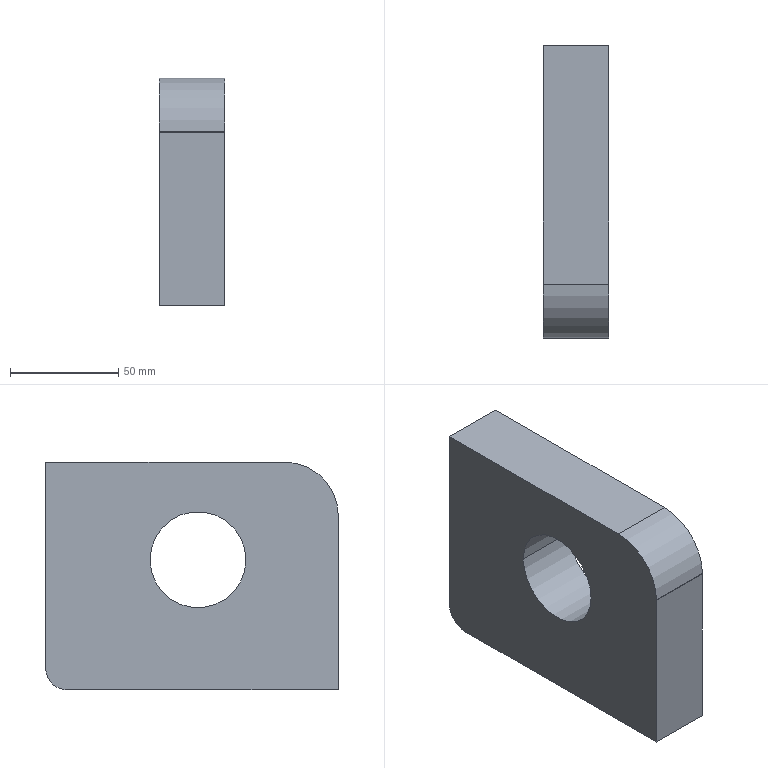Component | SolidWorks | ForkLug-1 | 1 solid | 11 faces | box 30 x 134.85 x 105 mm | volume 374154 mm3 | plane 6 | cylinder 5 | commonest cylinder face diameters 44.2 x2 49.483 x2 20 x1 | material Q235
build123d program:
from build123d import *

# Parameters (mm, degrees)
SKETCH1_R           = 22.1
BOSS_EXTRUDE1_DEPTH = 30


with BuildPart() as part:
    # Sketch1 → Boss-Extrude1 (new body)
    with BuildSketch(Plane.XY):
        with BuildLine():
            Line((3.712, 96.226), (103.712, 96.226))
            Line((103.712, 96.226), (113.712, 96.226))
            Line((113.712, 96.226), (113.712, 1.226))
            ThreePointArc((113.712, 1.226), (110.783, -5.845), (103.712, -8.774))
            Line((103.712, -8.774), (93.712, -8.774))
            Line((93.712, -8.774), (-21.136, -8.774))
            Line((-21.136, -8.774), (-21.136, 71.226))
            ThreePointArc((-21.136, 71.226), (-13.944, 88.926), (3.712, 96.226))
        make_face()
        with Locations((43.545, 51.226)):
            Circle(SKETCH1_R, mode=Mode.SUBTRACT)
    extrude(amount=BOSS_EXTRUDE1_DEPTH)


solid = part.part

# Placed as in the assembly
solid = solid.moved(Location((-1146.164, 1663.762, 2829.479), (90, 90, 0)))
STEP:
#1=COLOUR_RGB('',0.7922,0.8196,0.9333);
#2=FILL_AREA_STYLE_COLOUR('',#1);
#3=FILL_AREA_STYLE('',(#2));
#4=SURFACE_STYLE_FILL_AREA(#3);
#5=SURFACE_SIDE_STYLE('',(#4));
#6=SURFACE_STYLE_USAGE(.BOTH.,#5);
#7=PRESENTATION_STYLE_ASSIGNMENT((#6));
#8=CARTESIAN_POINT('',(-43.943,66.347,113.414));
#9=VERTEX_POINT('',#8);
#10=CARTESIAN_POINT('',(-43.943,68.087,113.414));
#11=VERTEX_POINT('',#10);
#12=CARTESIAN_POINT('',(-43.943,67.217,113.414));
#13=DIRECTION('',(1.,0.,-0.));
#14=DIRECTION('',(0.,1.,0.));
#15=AXIS2_PLACEMENT_3D('',#12,#13,#14);
#16=CIRCLE('',#15,0.8701);
#17=EDGE_CURVE('',#9,#11,#16,.T.);
#18=ORIENTED_EDGE('',*,*,#17,.T.);
#19=CARTESIAN_POINT('',(-45.125,68.087,113.414));
#20=VERTEX_POINT('',#19);
#21=CARTESIAN_POINT('',(-43.943,68.087,113.414));
#22=DIRECTION('',(-1.,-0.,0.));
#23=VECTOR('',#22,39.37);
#24=LINE('',#21,#23);
#25=EDGE_CURVE('',#11,#20,#24,.T.);
#26=ORIENTED_EDGE('',*,*,#25,.T.);
#27=CARTESIAN_POINT('',(-45.125,66.347,113.414));
#28=VERTEX_POINT('',#27);
#29=CARTESIAN_POINT('',(-45.125,67.217,113.414));
#30=DIRECTION('',(1.,0.,-0.));
#31=DIRECTION('',(0.,1.,0.));
#32=AXIS2_PLACEMENT_3D('',#29,#30,#31);
#33=CIRCLE('',#32,0.8701);
#34=EDGE_CURVE('',#28,#20,#33,.T.);
#35=ORIENTED_EDGE('',*,*,#34,.F.);
#36=CARTESIAN_POINT('',(-43.943,66.347,113.414));
#37=DIRECTION('',(-1.,-0.,0.));
#38=VECTOR('',#37,39.37);
#39=LINE('',#36,#38);
#40=EDGE_CURVE('',#9,#28,#39,.T.);
#41=ORIENTED_EDGE('',*,*,#40,.F.);
#42=EDGE_LOOP('',(#18,#26,#35,#41));
#43=FACE_OUTER_BOUND('',#42,.T.);
#44=CARTESIAN_POINT('',(-43.943,67.217,113.414));
#45=DIRECTION('',(-1.,-0.,0.));
#46=DIRECTION('',(0.,-1.,0.));
#47=AXIS2_PLACEMENT_3D('',#44,#45,#46);
#48=CYLINDRICAL_SURFACE('',#47,0.8701);
#49=ADVANCED_FACE('',(#43),#48,.F.);
#50=CARTESIAN_POINT('',(-43.943,64.67,114.211));
#51=VERTEX_POINT('',#50);
#52=CARTESIAN_POINT('',(-43.943,64.67,114.201));
#53=VERTEX_POINT('',#52);
#54=CARTESIAN_POINT('',(-43.943,65.644,114.211));
#55=DIRECTION('',(1.,0.,-0.));
#56=DIRECTION('',(0.,1.,0.));
#57=AXIS2_PLACEMENT_3D('',#54,#55,#56);
#58=CIRCLE('',#57,0.9741);
#59=EDGE_CURVE('',#51,#53,#58,.T.);
#60=ORIENTED_EDGE('',*,*,#59,.F.);
#61=CARTESIAN_POINT('',(-45.125,64.67,114.211));
#62=VERTEX_POINT('',#61);
#63=CARTESIAN_POINT('',(-43.943,64.67,114.211));
#64=DIRECTION('',(-1.,-0.,0.));
#65=VECTOR('',#64,39.37);
#66=LINE('',#63,#65);
#67=EDGE_CURVE('',#51,#62,#66,.T.);
#68=ORIENTED_EDGE('',*,*,#67,.T.);
#69=CARTESIAN_POINT('',(-45.125,64.67,114.201));
#70=VERTEX_POINT('',#69);
#71=CARTESIAN_POINT('',(-45.125,65.644,114.211));
#72=DIRECTION('',(1.,0.,-0.));
#73=DIRECTION('',(0.,1.,0.));
#74=AXIS2_PLACEMENT_3D('',#71,#72,#73);
#75=CIRCLE('',#74,0.9741);
#76=EDGE_CURVE('',#62,#70,#75,.T.);
#77=ORIENTED_EDGE('',*,*,#76,.T.);
#78=CARTESIAN_POINT('',(-43.943,64.67,114.201));
#79=DIRECTION('',(-1.,-0.,0.));
#80=VECTOR('',#79,39.37);
#81=LINE('',#78,#80);
#82=EDGE_CURVE('',#53,#70,#81,.T.);
#83=ORIENTED_EDGE('',*,*,#82,.F.);
#84=EDGE_LOOP('',(#60,#68,#77,#83));
#85=FACE_OUTER_BOUND('',#84,.T.);
#86=CARTESIAN_POINT('',(-43.943,65.644,114.211));
#87=DIRECTION('',(-1.,-0.,0.));
#88=DIRECTION('',(0.,-1.,0.));
#89=AXIS2_PLACEMENT_3D('',#86,#87,#88);
#90=CYLINDRICAL_SURFACE('',#89,0.9741);
#91=ADVANCED_FACE('',(#85),#90,.T.);
#92=CARTESIAN_POINT('',(-43.943,69.586,111.051));
#93=VERTEX_POINT('',#92);
#94=CARTESIAN_POINT('',(-43.943,69.979,111.445));
#95=VERTEX_POINT('',#94);
#96=CARTESIAN_POINT('',(-43.943,69.586,111.445));
#97=DIRECTION('',(1.,0.,-0.));
#98=DIRECTION('',(0.,1.,0.));
#99=AXIS2_PLACEMENT_3D('',#96,#97,#98);
#100=CIRCLE('',#99,0.3937);
#101=EDGE_CURVE('',#93,#95,#100,.T.);
#102=ORIENTED_EDGE('',*,*,#101,.T.);
#103=CARTESIAN_POINT('',(-43.943,69.979,115.185));
#104=VERTEX_POINT('',#103);
#105=CARTESIAN_POINT('',(-43.943,69.979,115.185));
#106=DIRECTION('',(0.,-0.,1.));
#107=VECTOR('',#106,39.37);
#108=LINE('',#105,#107);
#109=EDGE_CURVE('',#95,#104,#108,.T.);
#110=ORIENTED_EDGE('',*,*,#109,.T.);
#111=CARTESIAN_POINT('',(-43.943,65.649,115.185));
#112=VERTEX_POINT('',#111);
#113=CARTESIAN_POINT('',(-43.943,69.586,115.185));
#114=DIRECTION('',(0.,-1.,0.));
#115=VECTOR('',#114,39.37);
#116=LINE('',#113,#115);
#117=EDGE_CURVE('',#104,#112,#116,.T.);
#118=ORIENTED_EDGE('',*,*,#117,.T.);
#119=CARTESIAN_POINT('',(-43.943,65.644,114.211));
#120=DIRECTION('',(1.,0.,-0.));
#121=DIRECTION('',(0.,1.,0.));
#122=AXIS2_PLACEMENT_3D('',#119,#120,#121);
#123=CIRCLE('',#122,0.9741);
#124=EDGE_CURVE('',#112,#51,#123,.T.);
#125=ORIENTED_EDGE('',*,*,#124,.T.);
#126=ORIENTED_EDGE('',*,*,#59,.T.);
#127=CARTESIAN_POINT('',(-43.943,64.67,111.051));
#128=VERTEX_POINT('',#127);
#129=CARTESIAN_POINT('',(-43.943,64.67,114.201));
#130=DIRECTION('',(-0.,-0.,-1.));
#131=VECTOR('',#130,39.37);
#132=LINE('',#129,#131);
#133=EDGE_CURVE('',#53,#128,#132,.T.);
#134=ORIENTED_EDGE('',*,*,#133,.T.);
#135=CARTESIAN_POINT('',(-43.943,64.67,111.051));
#136=DIRECTION('',(-0.,1.,0.));
#137=VECTOR('',#136,39.37);
#138=LINE('',#135,#137);
#139=EDGE_CURVE('',#128,#93,#138,.T.);
#140=ORIENTED_EDGE('',*,*,#139,.T.);
#141=EDGE_LOOP('',(#102,#110,#118,#125,#126,#134,#140));
#142=FACE_OUTER_BOUND('',#141,.T.);
#143=ORIENTED_EDGE('',*,*,#17,.F.);
#144=CARTESIAN_POINT('',(-43.943,67.217,113.414));
#145=DIRECTION('',(1.,0.,-0.));
#146=DIRECTION('',(0.,1.,0.));
#147=AXIS2_PLACEMENT_3D('',#144,#145,#146);
#148=CIRCLE('',#147,0.8701);
#149=EDGE_CURVE('',#11,#9,#148,.T.);
#150=ORIENTED_EDGE('',*,*,#149,.F.);
#151=EDGE_LOOP('',(#143,#150));
#152=FACE_BOUND('',#151,.T.);
#153=CARTESIAN_POINT('',(-43.943,69.586,111.445));
#154=DIRECTION('',(1.,0.,-0.));
#155=DIRECTION('',(-0.,1.,0.));
#156=AXIS2_PLACEMENT_3D('',#153,#154,#155);
#157=PLANE('',#156);
#158=ADVANCED_FACE('',(#142,#152),#157,.T.);
#159=CARTESIAN_POINT('',(-45.125,69.586,111.051));
#160=VERTEX_POINT('',#159);
#161=CARTESIAN_POINT('',(-45.125,69.979,111.445));
#162=VERTEX_POINT('',#161);
#163=CARTESIAN_POINT('',(-45.125,69.586,111.445));
#164=DIRECTION('',(1.,0.,-0.));
#165=DIRECTION('',(0.,1.,0.));
#166=AXIS2_PLACEMENT_3D('',#163,#164,#165);
#167=CIRCLE('',#166,0.3937);
#168=EDGE_CURVE('',#160,#162,#167,.T.);
#169=ORIENTED_EDGE('',*,*,#168,.F.);
#170=CARTESIAN_POINT('',(-45.125,64.67,111.051));
#171=VERTEX_POINT('',#170);
#172=CARTESIAN_POINT('',(-45.125,69.192,111.051));
#173=DIRECTION('',(-0.,1.,0.));
#174=VECTOR('',#173,39.37);
#175=LINE('',#172,#174);
#176=EDGE_CURVE('',#171,#160,#175,.T.);
#177=ORIENTED_EDGE('',*,*,#176,.F.);
#178=CARTESIAN_POINT('',(-45.125,64.67,114.201));
#179=DIRECTION('',(-0.,-0.,-1.));
#180=VECTOR('',#179,39.37);
#181=LINE('',#178,#180);
#182=EDGE_CURVE('',#70,#171,#181,.T.);
#183=ORIENTED_EDGE('',*,*,#182,.F.);
#184=ORIENTED_EDGE('',*,*,#76,.F.);
#185=CARTESIAN_POINT('',(-45.125,65.649,115.185));
#186=VERTEX_POINT('',#185);
#187=CARTESIAN_POINT('',(-45.125,65.644,114.211));
#188=DIRECTION('',(1.,0.,-0.));
#189=DIRECTION('',(0.,1.,0.));
#190=AXIS2_PLACEMENT_3D('',#187,#188,#189);
#191=CIRCLE('',#190,0.9741);
#192=EDGE_CURVE('',#186,#62,#191,.T.);
#193=ORIENTED_EDGE('',*,*,#192,.F.);
#194=CARTESIAN_POINT('',(-45.125,69.979,115.185));
#195=VERTEX_POINT('',#194);
#196=CARTESIAN_POINT('',(-45.125,65.649,115.185));
#197=DIRECTION('',(0.,-1.,0.));
#198=VECTOR('',#197,39.37);
#199=LINE('',#196,#198);
#200=EDGE_CURVE('',#195,#186,#199,.T.);
#201=ORIENTED_EDGE('',*,*,#200,.F.);
#202=CARTESIAN_POINT('',(-45.125,69.979,115.185));
#203=DIRECTION('',(0.,-0.,1.));
#204=VECTOR('',#203,39.37);
#205=LINE('',#202,#204);
#206=EDGE_CURVE('',#162,#195,#205,.T.);
#207=ORIENTED_EDGE('',*,*,#206,.F.);
#208=EDGE_LOOP('',(#169,#177,#183,#184,#193,#201,#207));
#209=FACE_OUTER_BOUND('',#208,.T.);
#210=ORIENTED_EDGE('',*,*,#34,.T.);
#211=CARTESIAN_POINT('',(-45.125,67.217,113.414));
#212=DIRECTION('',(1.,0.,-0.));
#213=DIRECTION('',(0.,1.,0.));
#214=AXIS2_PLACEMENT_3D('',#211,#212,#213);
#215=CIRCLE('',#214,0.8701);
#216=EDGE_CURVE('',#20,#28,#215,.T.);
#217=ORIENTED_EDGE('',*,*,#216,.T.);
#218=EDGE_LOOP('',(#210,#217));
#219=FACE_BOUND('',#218,.T.);
#220=CARTESIAN_POINT('',(-45.125,69.586,111.445));
#221=DIRECTION('',(1.,0.,-0.));
#222=DIRECTION('',(-0.,1.,0.));
#223=AXIS2_PLACEMENT_3D('',#220,#221,#222);
#224=PLANE('',#223);
#225=ADVANCED_FACE('',(#209,#219),#224,.F.);
#226=ORIENTED_EDGE('',*,*,#168,.T.);
#227=CARTESIAN_POINT('',(-43.943,69.979,111.445));
#228=DIRECTION('',(-1.,-0.,0.));
#229=VECTOR('',#228,39.37);
#230=LINE('',#227,#229);
#231=EDGE_CURVE('',#95,#162,#230,.T.);
#232=ORIENTED_EDGE('',*,*,#231,.F.);
#233=ORIENTED_EDGE('',*,*,#101,.F.);
#234=CARTESIAN_POINT('',(-43.943,69.586,111.051));
#235=DIRECTION('',(-1.,-0.,0.));
#236=VECTOR('',#235,39.37);
#237=LINE('',#234,#236);
#238=EDGE_CURVE('',#93,#160,#237,.T.);
#239=ORIENTED_EDGE('',*,*,#238,.T.);
#240=EDGE_LOOP('',(#226,#232,#233,#239));
#241=FACE_OUTER_BOUND('',#240,.T.);
#242=CARTESIAN_POINT('',(-43.943,69.586,111.445));
#243=DIRECTION('',(-1.,-0.,0.));
#244=DIRECTION('',(0.,-1.,0.));
#245=AXIS2_PLACEMENT_3D('',#242,#243,#244);
#246=CYLINDRICAL_SURFACE('',#245,0.3937);
#247=ADVANCED_FACE('',(#241),#246,.T.);
#248=ORIENTED_EDGE('',*,*,#206,.T.);
#249=CARTESIAN_POINT('',(-43.943,69.979,115.185));
#250=DIRECTION('',(-1.,-0.,0.));
#251=VECTOR('',#250,39.37);
#252=LINE('',#249,#251);
#253=EDGE_CURVE('',#104,#195,#252,.T.);
#254=ORIENTED_EDGE('',*,*,#253,.F.);
#255=ORIENTED_EDGE('',*,*,#109,.F.);
#256=ORIENTED_EDGE('',*,*,#231,.T.);
#257=EDGE_LOOP('',(#248,#254,#255,#256));
#258=FACE_OUTER_BOUND('',#257,.T.);
#259=CARTESIAN_POINT('',(-43.943,69.979,115.185));
#260=DIRECTION('',(0.,-1.,-0.));
#261=DIRECTION('',(1.,0.,-0.));
#262=AXIS2_PLACEMENT_3D('',#259,#260,#261);
#263=PLANE('',#262);
#264=ADVANCED_FACE('',(#258),#263,.F.);
#265=ORIENTED_EDGE('',*,*,#200,.T.);
#266=CARTESIAN_POINT('',(-43.943,65.649,115.185));
#267=DIRECTION('',(-1.,-0.,0.));
#268=VECTOR('',#267,39.37);
#269=LINE('',#266,#268);
#270=EDGE_CURVE('',#112,#186,#269,.T.);
#271=ORIENTED_EDGE('',*,*,#270,.F.);
#272=ORIENTED_EDGE('',*,*,#117,.F.);
#273=ORIENTED_EDGE('',*,*,#253,.T.);
#274=EDGE_LOOP('',(#265,#271,#272,#273));
#275=FACE_OUTER_BOUND('',#274,.T.);
#276=CARTESIAN_POINT('',(-43.943,65.649,115.185));
#277=DIRECTION('',(-0.,0.,-1.));
#278=DIRECTION('',(-1.,-0.,0.));
#279=AXIS2_PLACEMENT_3D('',#276,#277,#278);
#280=PLANE('',#279);
#281=ADVANCED_FACE('',(#275),#280,.F.);
#282=ORIENTED_EDGE('',*,*,#67,.F.);
#283=ORIENTED_EDGE('',*,*,#124,.F.);
#284=ORIENTED_EDGE('',*,*,#270,.T.);
#285=ORIENTED_EDGE('',*,*,#192,.T.);
#286=EDGE_LOOP('',(#282,#283,#284,#285));
#287=FACE_OUTER_BOUND('',#286,.T.);
#288=CARTESIAN_POINT('',(-43.943,65.644,114.211));
#289=DIRECTION('',(-1.,-0.,0.));
#290=DIRECTION('',(0.,-1.,0.));
#291=AXIS2_PLACEMENT_3D('',#288,#289,#290);
#292=CYLINDRICAL_SURFACE('',#291,0.9741);
#293=ADVANCED_FACE('',(#287),#292,.T.);
#294=ORIENTED_EDGE('',*,*,#182,.T.);
#295=CARTESIAN_POINT('',(-43.943,64.67,111.051));
#296=DIRECTION('',(-1.,-0.,0.));
#297=VECTOR('',#296,39.37);
#298=LINE('',#295,#297);
#299=EDGE_CURVE('',#128,#171,#298,.T.);
#300=ORIENTED_EDGE('',*,*,#299,.F.);
#301=ORIENTED_EDGE('',*,*,#133,.F.);
#302=ORIENTED_EDGE('',*,*,#82,.T.);
#303=EDGE_LOOP('',(#294,#300,#301,#302));
#304=FACE_OUTER_BOUND('',#303,.T.);
#305=CARTESIAN_POINT('',(-43.943,64.67,114.201));
#306=DIRECTION('',(-0.,1.,-0.));
#307=DIRECTION('',(0.,0.,1.));
#308=AXIS2_PLACEMENT_3D('',#305,#306,#307);
#309=PLANE('',#308);
#310=ADVANCED_FACE('',(#304),#309,.F.);
#311=ORIENTED_EDGE('',*,*,#176,.T.);
#312=ORIENTED_EDGE('',*,*,#238,.F.);
#313=ORIENTED_EDGE('',*,*,#139,.F.);
#314=ORIENTED_EDGE('',*,*,#299,.T.);
#315=EDGE_LOOP('',(#311,#312,#313,#314));
#316=FACE_OUTER_BOUND('',#315,.T.);
#317=CARTESIAN_POINT('',(-43.943,69.192,111.051));
#318=DIRECTION('',(0.,-0.,1.));
#319=DIRECTION('',(1.,0.,-0.));
#320=AXIS2_PLACEMENT_3D('',#317,#318,#319);
#321=PLANE('',#320);
#322=ADVANCED_FACE('',(#316),#321,.F.);
#323=ORIENTED_EDGE('',*,*,#25,.F.);
#324=ORIENTED_EDGE('',*,*,#149,.T.);
#325=ORIENTED_EDGE('',*,*,#40,.T.);
#326=ORIENTED_EDGE('',*,*,#216,.F.);
#327=EDGE_LOOP('',(#323,#324,#325,#326));
#328=FACE_OUTER_BOUND('',#327,.T.);
#329=CARTESIAN_POINT('',(-43.943,67.217,113.414));
#330=DIRECTION('',(-1.,-0.,0.));
#331=DIRECTION('',(0.,-1.,0.));
#332=AXIS2_PLACEMENT_3D('',#329,#330,#331);
#333=CYLINDRICAL_SURFACE('',#332,0.8701);
#334=ADVANCED_FACE('',(#328),#333,.F.);
#335=CLOSED_SHELL('',(#49,#91,#158,#225,#247,#264,#281,#293,#310,#322,#334));
#336=MANIFOLD_SOLID_BREP('',#335);
#337=STYLED_ITEM('',(#7),#336);
#338=(LENGTH_UNIT()NAMED_UNIT(*)SI_UNIT($,.METRE.));
#339=LENGTH_MEASURE_WITH_UNIT(LENGTH_MEASURE(0.0254),#338);
#340=DIMENSIONAL_EXPONENTS(1.,0.,0.,0.,0.,0.,0.);
#341=(CONVERSION_BASED_UNIT('',#339)LENGTH_UNIT()NAMED_UNIT(#340));
#342=UNCERTAINTY_MEASURE_WITH_UNIT(LENGTH_MEASURE(0.00001),#341,'','');
#343=(NAMED_UNIT(*)PLANE_ANGLE_UNIT()SI_UNIT($,.RADIAN.));
#344=(NAMED_UNIT(*)SI_UNIT($,.STERADIAN.)SOLID_ANGLE_UNIT());
#345=(GEOMETRIC_REPRESENTATION_CONTEXT(3)GLOBAL_UNCERTAINTY_ASSIGNED_CONTEXT((#342))GLOBAL_UNIT_ASSIGNED_CONTEXT((#341,#343,#344))REPRESENTATION_CONTEXT('',''));
#346=MECHANICAL_DESIGN_GEOMETRIC_PRESENTATION_REPRESENTATION('',(#337),#345);
#347=CARTESIAN_POINT('',(0.,0.,0.));
#348=DIRECTION('',(0.,0.,1.));
#349=DIRECTION('',(1.,0.,0.));
#350=AXIS2_PLACEMENT_3D('',#347,#348,#349);
#351=(LENGTH_UNIT()NAMED_UNIT(*)SI_UNIT($,.METRE.));
#352=LENGTH_MEASURE_WITH_UNIT(LENGTH_MEASURE(0.0254),#351);
#353=DIMENSIONAL_EXPONENTS(1.,0.,0.,0.,0.,0.,0.);
#354=(CONVERSION_BASED_UNIT('',#352)LENGTH_UNIT()NAMED_UNIT(#353));
#355=UNCERTAINTY_MEASURE_WITH_UNIT(LENGTH_MEASURE(0.00001),#354,'','');
#356=(NAMED_UNIT(*)PLANE_ANGLE_UNIT()SI_UNIT($,.RADIAN.));
#357=(NAMED_UNIT(*)SI_UNIT($,.STERADIAN.)SOLID_ANGLE_UNIT());
#358=(GEOMETRIC_REPRESENTATION_CONTEXT(3)GLOBAL_UNCERTAINTY_ASSIGNED_CONTEXT((#355))GLOBAL_UNIT_ASSIGNED_CONTEXT((#354,#356,#357))REPRESENTATION_CONTEXT('',''));
#359=ADVANCED_BREP_SHAPE_REPRESENTATION('',(#336,#350),#358);
#360=PRESENTATION_LAYER_ASSIGNMENT('','',(#337));